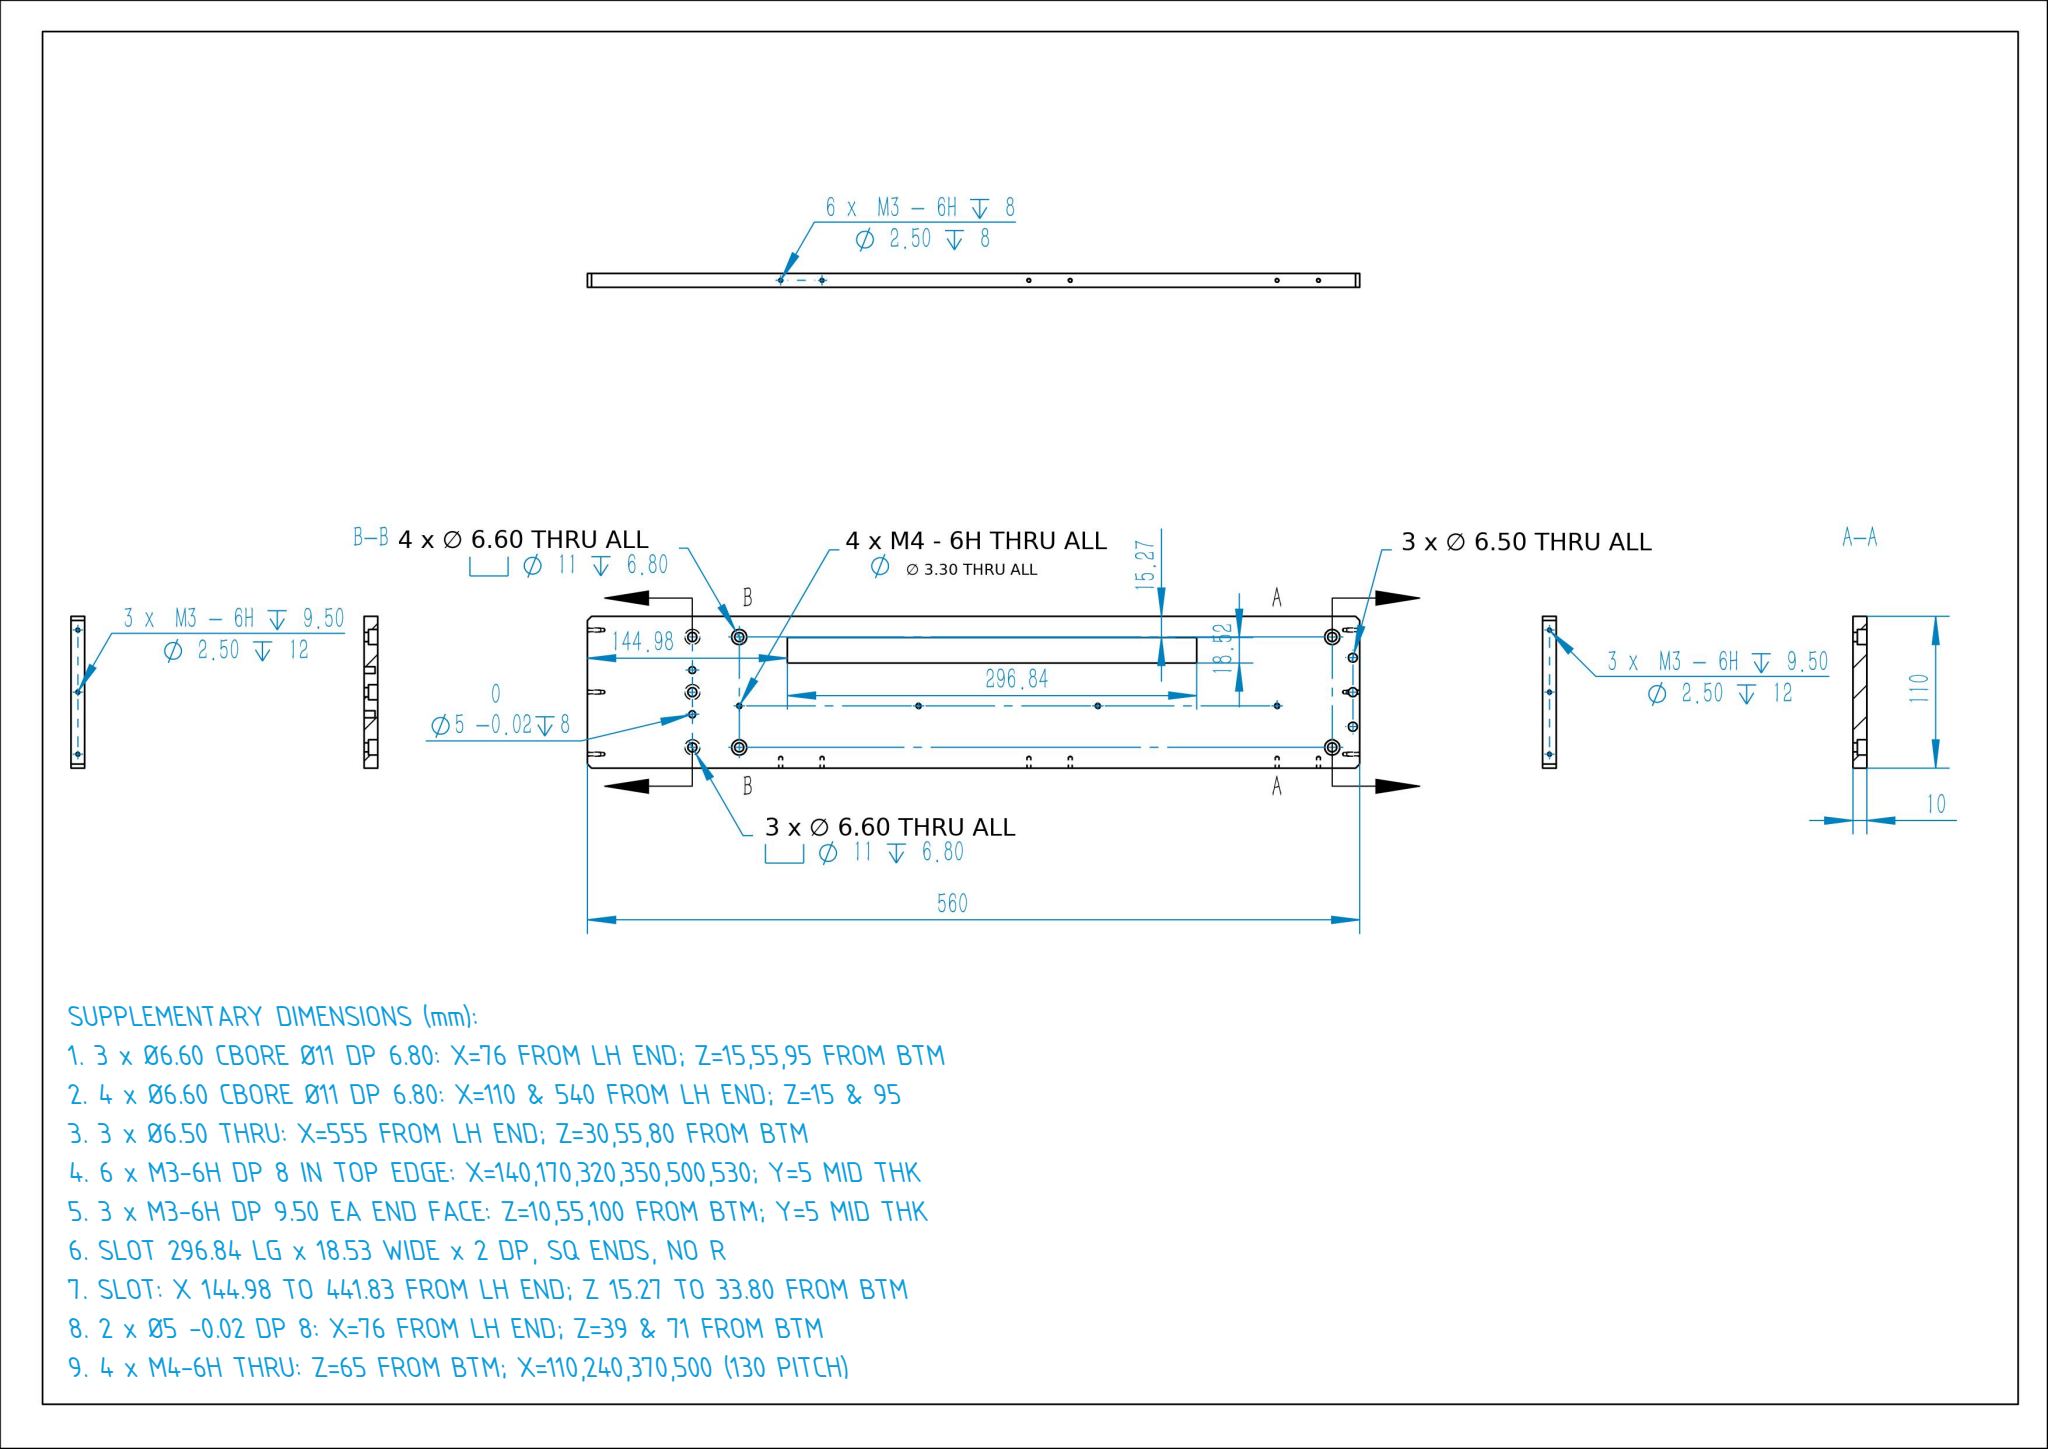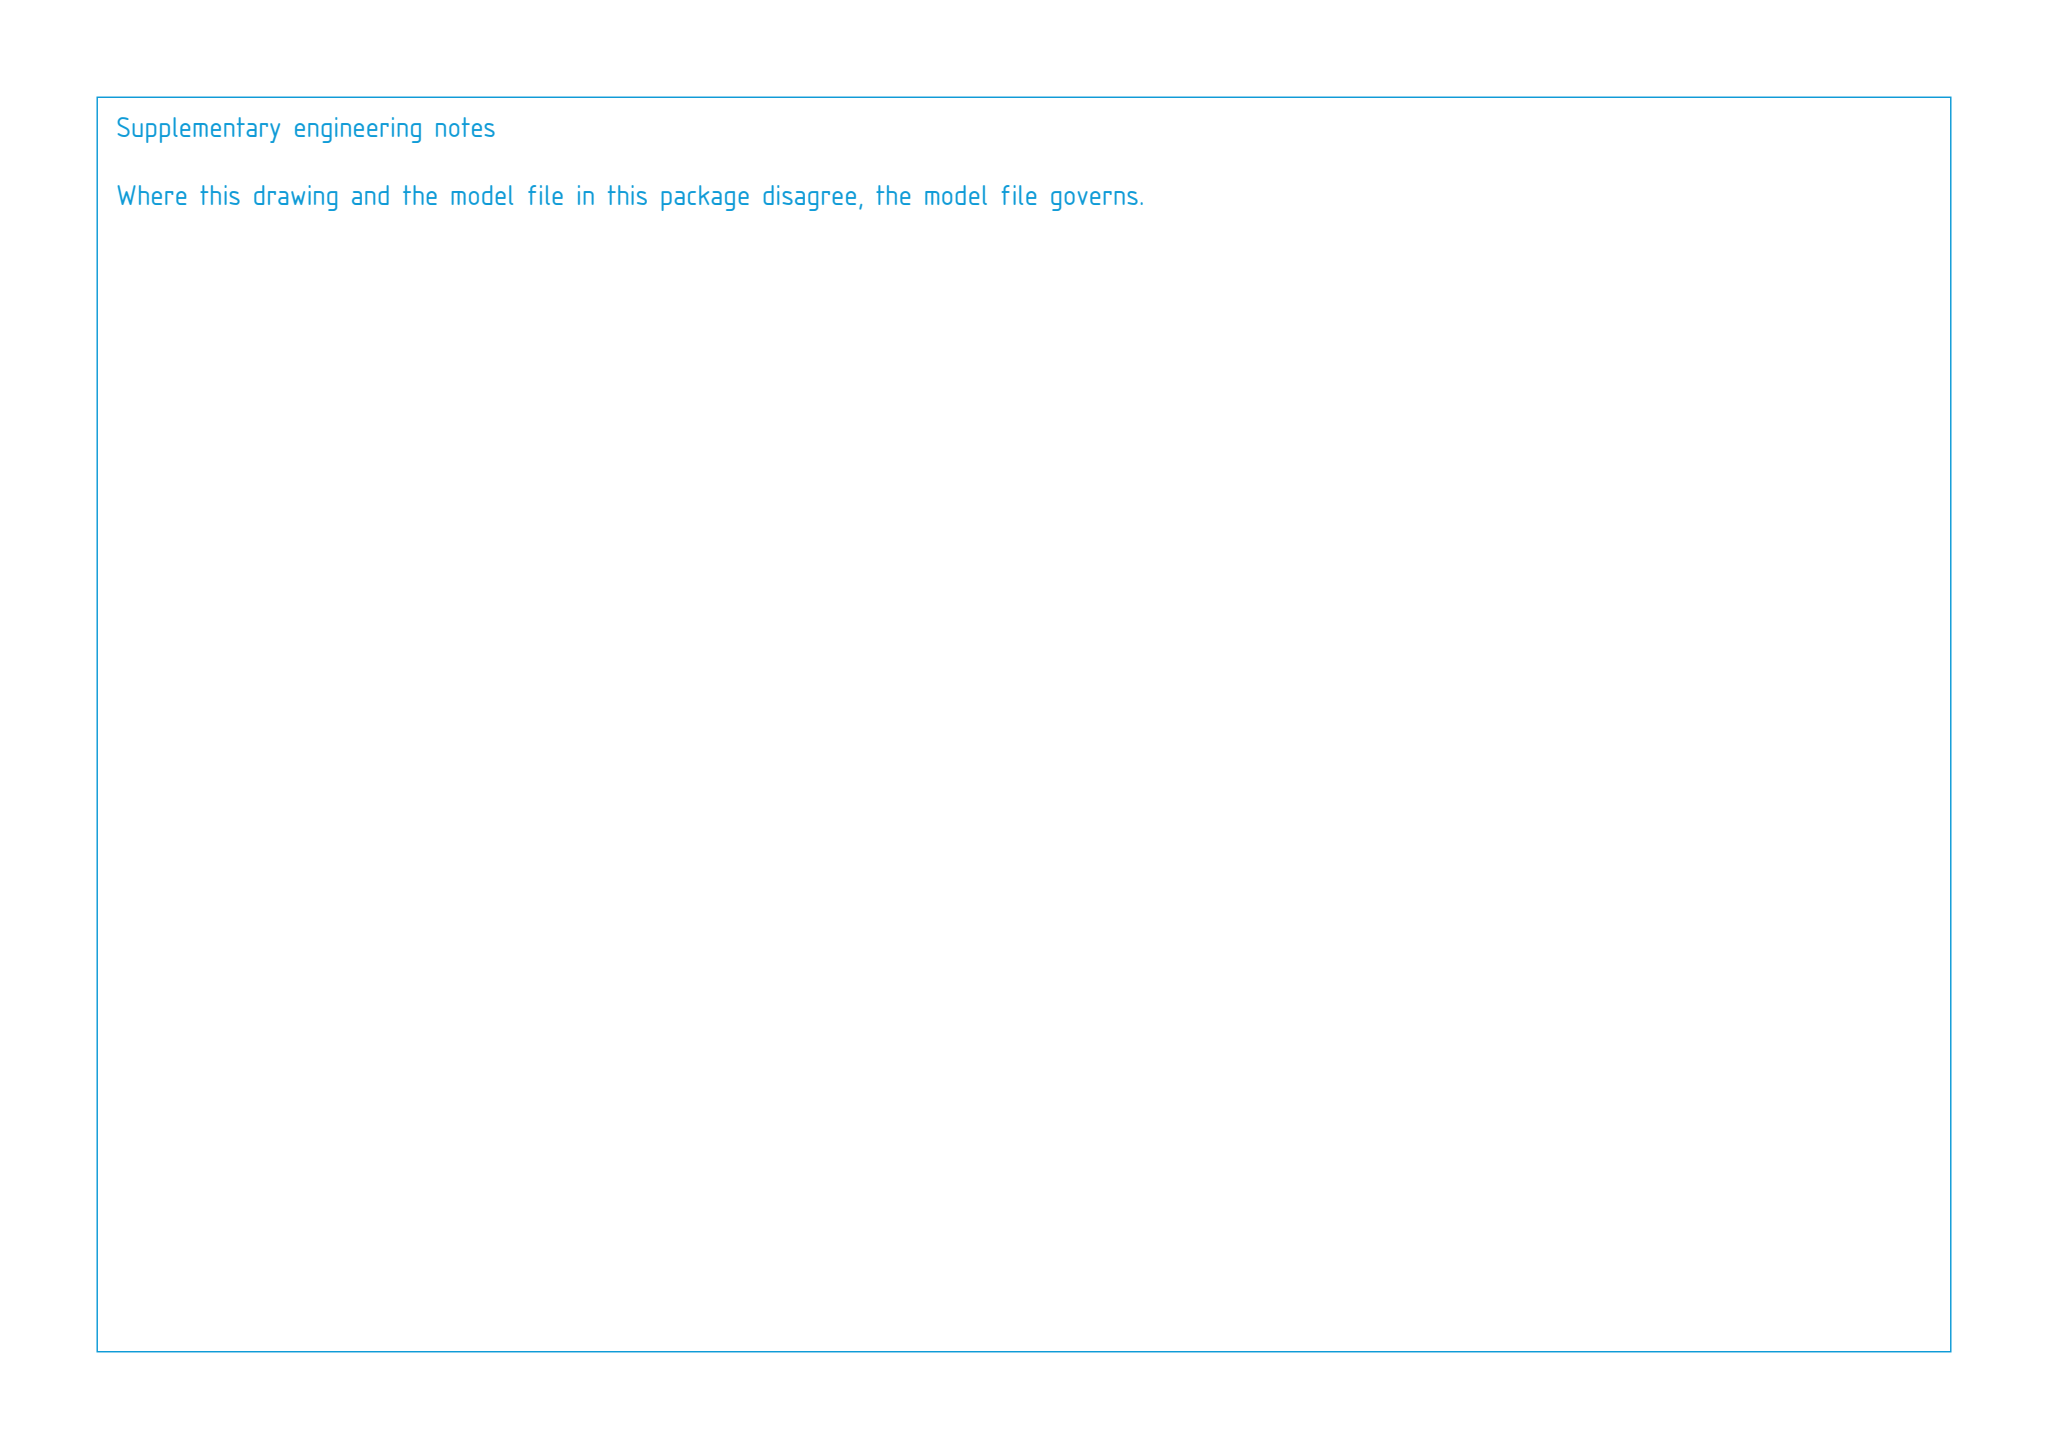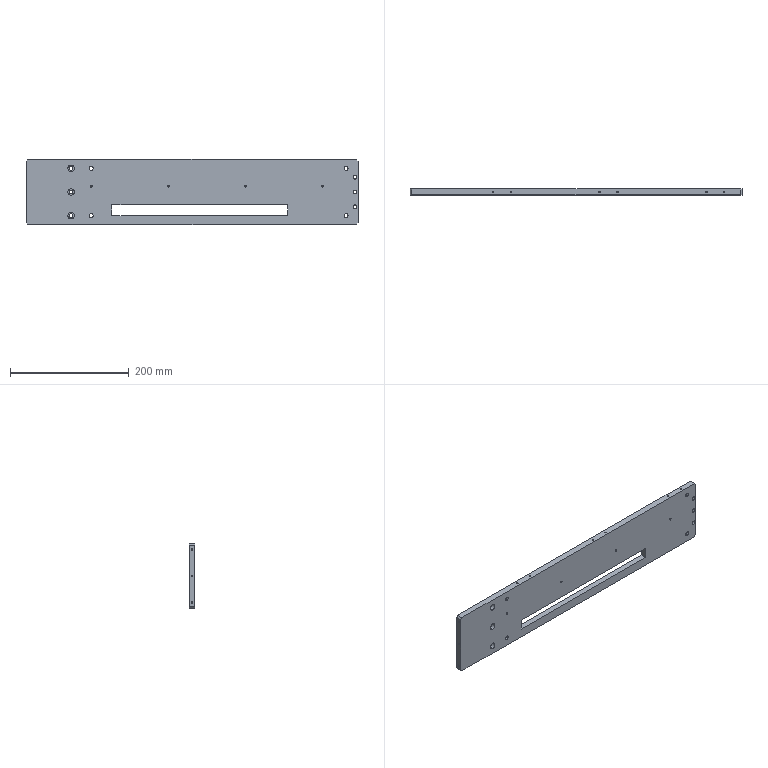Part | SolidWorks | mm | 1 solid | 119 faces | box 560 x 10 x 110 mm | volume 553324 mm3 | cylinder 72 | cone 24 | plane 23 | commonest cylinder face diameters 2.5 x26 6.6 x14 11 x14 3.3 x8 6.5 x6 5 x4
build123d program:
from build123d import *

# Parameters (mm, degrees)
SKETCH1_W                                            = 560
SKETCH1_H                                            = 110
BOSS_EXTRUDE1_DEPTH                                  = 5
HOLE_SIZE_ACCORDING_TO_HEXAGON_SOCKET_HE_D           = 6.6
HOLE_SIZE_ACCORDING_TO_HEXAGON_SOCKET_HE_CBORE_D     = 11
HOLE_SIZE_ACCORDING_TO_HEXAGON_SOCKET_HE_CBORE_DEPTH = 6.8
LPATTERN1_COUNT                                      = 2
LPATTERN1_PITCH                                      = 430
LPATTERN1_COUNT_DIR2                                 = 2
LPATTERN1_PITCH_DIR2                                 = 80
CHAMFER1_SIZE                                        = 3
HOLE_SIZE_ACCORDING_TO_HEXAGON_SOCKE_2_D             = 6.6
HOLE_SIZE_ACCORDING_TO_HEXAGON_SOCKE_2_CBORE_D       = 11
HOLE_SIZE_ACCORDING_TO_HEXAGON_SOCKE_2_CBORE_DEPTH   = 6.8
LPATTERN2_COUNT                                      = 3
LPATTERN2_PITCH                                      = 40
SKETCH6_R                                            = 2.5
CUT_EXTRUDE1_DEPTH                                   = 8
LPATTERN3_COUNT                                      = 2
LPATTERN3_PITCH                                      = 32
F_6_5_6_5_DIAMETER_HOLE1_D                           = 6.5
LPATTERN4_COUNT                                      = 3
LPATTERN4_PITCH                                      = 25
M4_TAPPED_HOLE1_D                                    = 3.3
LPATTERN7_COUNT                                      = 4
LPATTERN7_PITCH                                      = 130
LPATTERN8_COUNT                                      = 2
LPATTERN8_PITCH                                      = 30
LPATTERN9_COUNT                                      = 3
LPATTERN9_PITCH                                      = 180
LPATTERN10_COUNT                                     = 3
LPATTERN10_PITCH                                     = 45
SKETCH19_W                                           = 296.842
SKETCH19_H                                           = 18.522
CUT_EXTRUDE2_DEPTH                                   = 71


with BuildPart() as part:
    # Sketch1 → Boss-Extrude1 (new, symmetric)
    with BuildSketch(Plane(origin=(0, 0, 0), x_dir=(1, 0, 0), z_dir=(0, 1, 0))):
        Rectangle(SKETCH1_W, SKETCH1_H)
    extrude(amount=BOSS_EXTRUDE1_DEPTH, both=True)

    # Hole Size according to Hexagon Socket He (through all)
    with Locations(Plane(origin=(0, 5, 0), x_dir=(1, 0, 0), z_dir=(0, 1, 0))):
        with Locations((-170, 40)):
            hole_size_according_to_hexagon_socket_he = CounterBoreHole(HOLE_SIZE_ACCORDING_TO_HEXAGON_SOCKET_HE_D / 2, HOLE_SIZE_ACCORDING_TO_HEXAGON_SOCKET_HE_CBORE_D / 2, HOLE_SIZE_ACCORDING_TO_HEXAGON_SOCKET_HE_CBORE_DEPTH)

    # LPattern1: Hole Size according to Hexagon Socket He 2 × 2
    with Locations(*[(i * LPATTERN1_PITCH, 0, j * LPATTERN1_PITCH_DIR2) for i in range(LPATTERN1_COUNT) for j in range(LPATTERN1_COUNT_DIR2) if (i, j) != (0, 0)]):
        add(hole_size_according_to_hexagon_socket_he, mode=Mode.SUBTRACT)

    # Chamfer1
    chamfer1_edges = [part.edges().sort_by_distance(p)[0] for p in [
        (280, 0, 55),
        (-280, 0, 55),
        (-280, 0, -55),
        (280, 0, -55),
    ]]
    chamfer(chamfer1_edges, length=CHAMFER1_SIZE)

    # Hole Size according to Hexagon Socke 2 (through all)
    with Locations(Plane(origin=(0, -5, 0), x_dir=(-1, 0, 0), z_dir=(0, -1, 0))):
        with Locations((204, 40)):
            hole_size_according_to_hexagon_socke_2 = CounterBoreHole(HOLE_SIZE_ACCORDING_TO_HEXAGON_SOCKE_2_D / 2, HOLE_SIZE_ACCORDING_TO_HEXAGON_SOCKE_2_CBORE_D / 2, HOLE_SIZE_ACCORDING_TO_HEXAGON_SOCKE_2_CBORE_DEPTH)

    # LPattern2: Hole Size according to Hexagon Socke 2 ×3
    with Locations(*[(0, 0, i * LPATTERN2_PITCH) for i in range(1, LPATTERN2_COUNT)]):
        add(hole_size_according_to_hexagon_socke_2, mode=Mode.SUBTRACT)

    # Sketch6 → Cut-Extrude1 (cut)
    with BuildSketch(Plane(origin=(0, 5, 0), x_dir=(1, 0, 0), z_dir=(0, 1, 0))):
        with Locations(Location((-204, 16, 0), (0, 0, 270))):
            Circle(SKETCH6_R)
    cut_extrude1 = extrude(amount=-CUT_EXTRUDE1_DEPTH, mode=Mode.SUBTRACT)

    # LPattern3: Cut-Extrude1 ×2
    with Locations(*[(0, 0, i * LPATTERN3_PITCH) for i in range(1, LPATTERN3_COUNT)]):
        add(cut_extrude1, mode=Mode.SUBTRACT)

    # 6.5 _6.5_ Diameter Hole1 (through all)
    with Locations(Plane(origin=(0, -5, 0), x_dir=(-1, 0, 0), z_dir=(0, -1, 0))):
        with Locations((-275, -25)):
            f_6_5_6_5_diameter_hole1 = Hole(F_6_5_6_5_DIAMETER_HOLE1_D / 2)

    # LPattern4: 6.5 _6.5_ Diameter Hole1 ×3
    with Locations(*[(0, 0, -i * LPATTERN4_PITCH) for i in range(1, LPATTERN4_COUNT)]):
        add(f_6_5_6_5_diameter_hole1, mode=Mode.SUBTRACT)

    # M4 Tapped Hole1 (through all)
    with Locations(Plane(origin=(0, -5, 0), x_dir=(-1, 0, 0), z_dir=(0, -1, 0))):
        with Locations((-220, -10)):
            m4_tapped_hole1 = Hole(M4_TAPPED_HOLE1_D / 2)

    # LPattern7: M4 Tapped Hole1 ×4
    with Locations(*[(-i * LPATTERN7_PITCH, 0, 0) for i in range(1, LPATTERN7_COUNT)]):
        add(m4_tapped_hole1, mode=Mode.SUBTRACT)

    # Sketch15 → M3 Tapped Hole1 (revolve, cut)
    with BuildSketch(Plane(origin=(-140, 0, 55), x_dir=(0, -1, 0), z_dir=(1, 0, 0))):
        Polygon((0, 0), (0, 8.751), (1.25, 8), (1.25, 0), align=None)
    m3_tapped_hole1 = revolve(axis=Axis((-140, 0, 61.35), (0, 0, -1)), mode=Mode.SUBTRACT)

    # LPattern8: M3 Tapped Hole1 ×2
    with Locations(*[(i * LPATTERN8_PITCH, 0, 0) for i in range(1, LPATTERN8_COUNT)]):
        add(m3_tapped_hole1, mode=Mode.SUBTRACT)

    # LPattern9: M3 Tapped Hole1 ×3
    with Locations(*[(i * LPATTERN9_PITCH, 0, 0) for i in range(1, LPATTERN9_COUNT)]):
        add(m3_tapped_hole1, mode=Mode.SUBTRACT)

    # LPattern9 copy 1 sketch → LPattern9 copy 1 (revolve, cut)
    with BuildSketch(Plane(origin=(70, 0, 55), x_dir=(0, -1, 0), z_dir=(1, 0, 0))):
        Polygon((0, 0), (0, 8.751), (1.25, 8), (1.25, 0), align=None)
    revolve(axis=Axis((70, 0, 61.35), (0, 0, -1)), mode=Mode.SUBTRACT)

    # LPattern9 copy 2 sketch → LPattern9 copy 2 (revolve, cut)
    with BuildSketch(Plane(origin=(250, 0, 55), x_dir=(0, -1, 0), z_dir=(1, 0, 0))):
        Polygon((0, 0), (0, 8.751), (1.25, 8), (1.25, 0), align=None)
    revolve(axis=Axis((250, 0, 61.35), (0, 0, -1)), mode=Mode.SUBTRACT)

    # Sketch17 → M3 Tapped Hole2 (revolve, cut)
    with BuildSketch(Plane(origin=(-280, 0, -45), x_dir=(0, 0, 1), z_dir=(0, 1, 0))):
        Polygon((0, 0), (0, 12.751), (1.25, 12), (1.25, 0), align=None)
    m3_tapped_hole2 = revolve(axis=Axis((-286.35, 0, -45), (1, 0, 0)), mode=Mode.SUBTRACT)

    # LPattern10: M3 Tapped Hole2 ×3
    with Locations(*[(0, 0, i * LPATTERN10_PITCH) for i in range(1, LPATTERN10_COUNT)]):
        add(m3_tapped_hole2, mode=Mode.SUBTRACT)

    # Mirror1: M3 Tapped Hole2 across plane
    add(m3_tapped_hole2.mirror(Plane(origin=(0, 0, 0), x_dir=(0, 0, 1), z_dir=(1, 0, 0))), mode=Mode.SUBTRACT)

    # Mirror1 copy 1 sketch → Mirror1 copy 1 (revolve, cut)
    with BuildSketch(Plane(origin=(280, 0, 0), x_dir=(0, 0, 1), z_dir=(0, 1, 0))):
        Polygon((0, 0), (0, -12.751), (1.25, -12), (1.25, 0), align=None)
    revolve(axis=Axis((286.35, 0, 0), (1, 0, 0)), mode=Mode.SUBTRACT)

    # Mirror1 copy 2 sketch → Mirror1 copy 2 (revolve, cut)
    with BuildSketch(Plane(origin=(280, 0, 45), x_dir=(0, 0, 1), z_dir=(0, 1, 0))):
        Polygon((0, 0), (0, -12.751), (1.25, -12), (1.25, 0), align=None)
    revolve(axis=Axis((286.35, 0, 45), (1, 0, 0)), mode=Mode.SUBTRACT)

    # Sketch19 → Cut-Extrude2 (cut)
    with BuildSketch(Plane(origin=(0, 5, 0), x_dir=(1, 0, 0), z_dir=(0, 1, 0))):
        with Locations((13.404, 30.464)):
            Rectangle(SKETCH19_W, SKETCH19_H)
    extrude(amount=-CUT_EXTRUDE2_DEPTH, mode=Mode.SUBTRACT)


solid = part.part